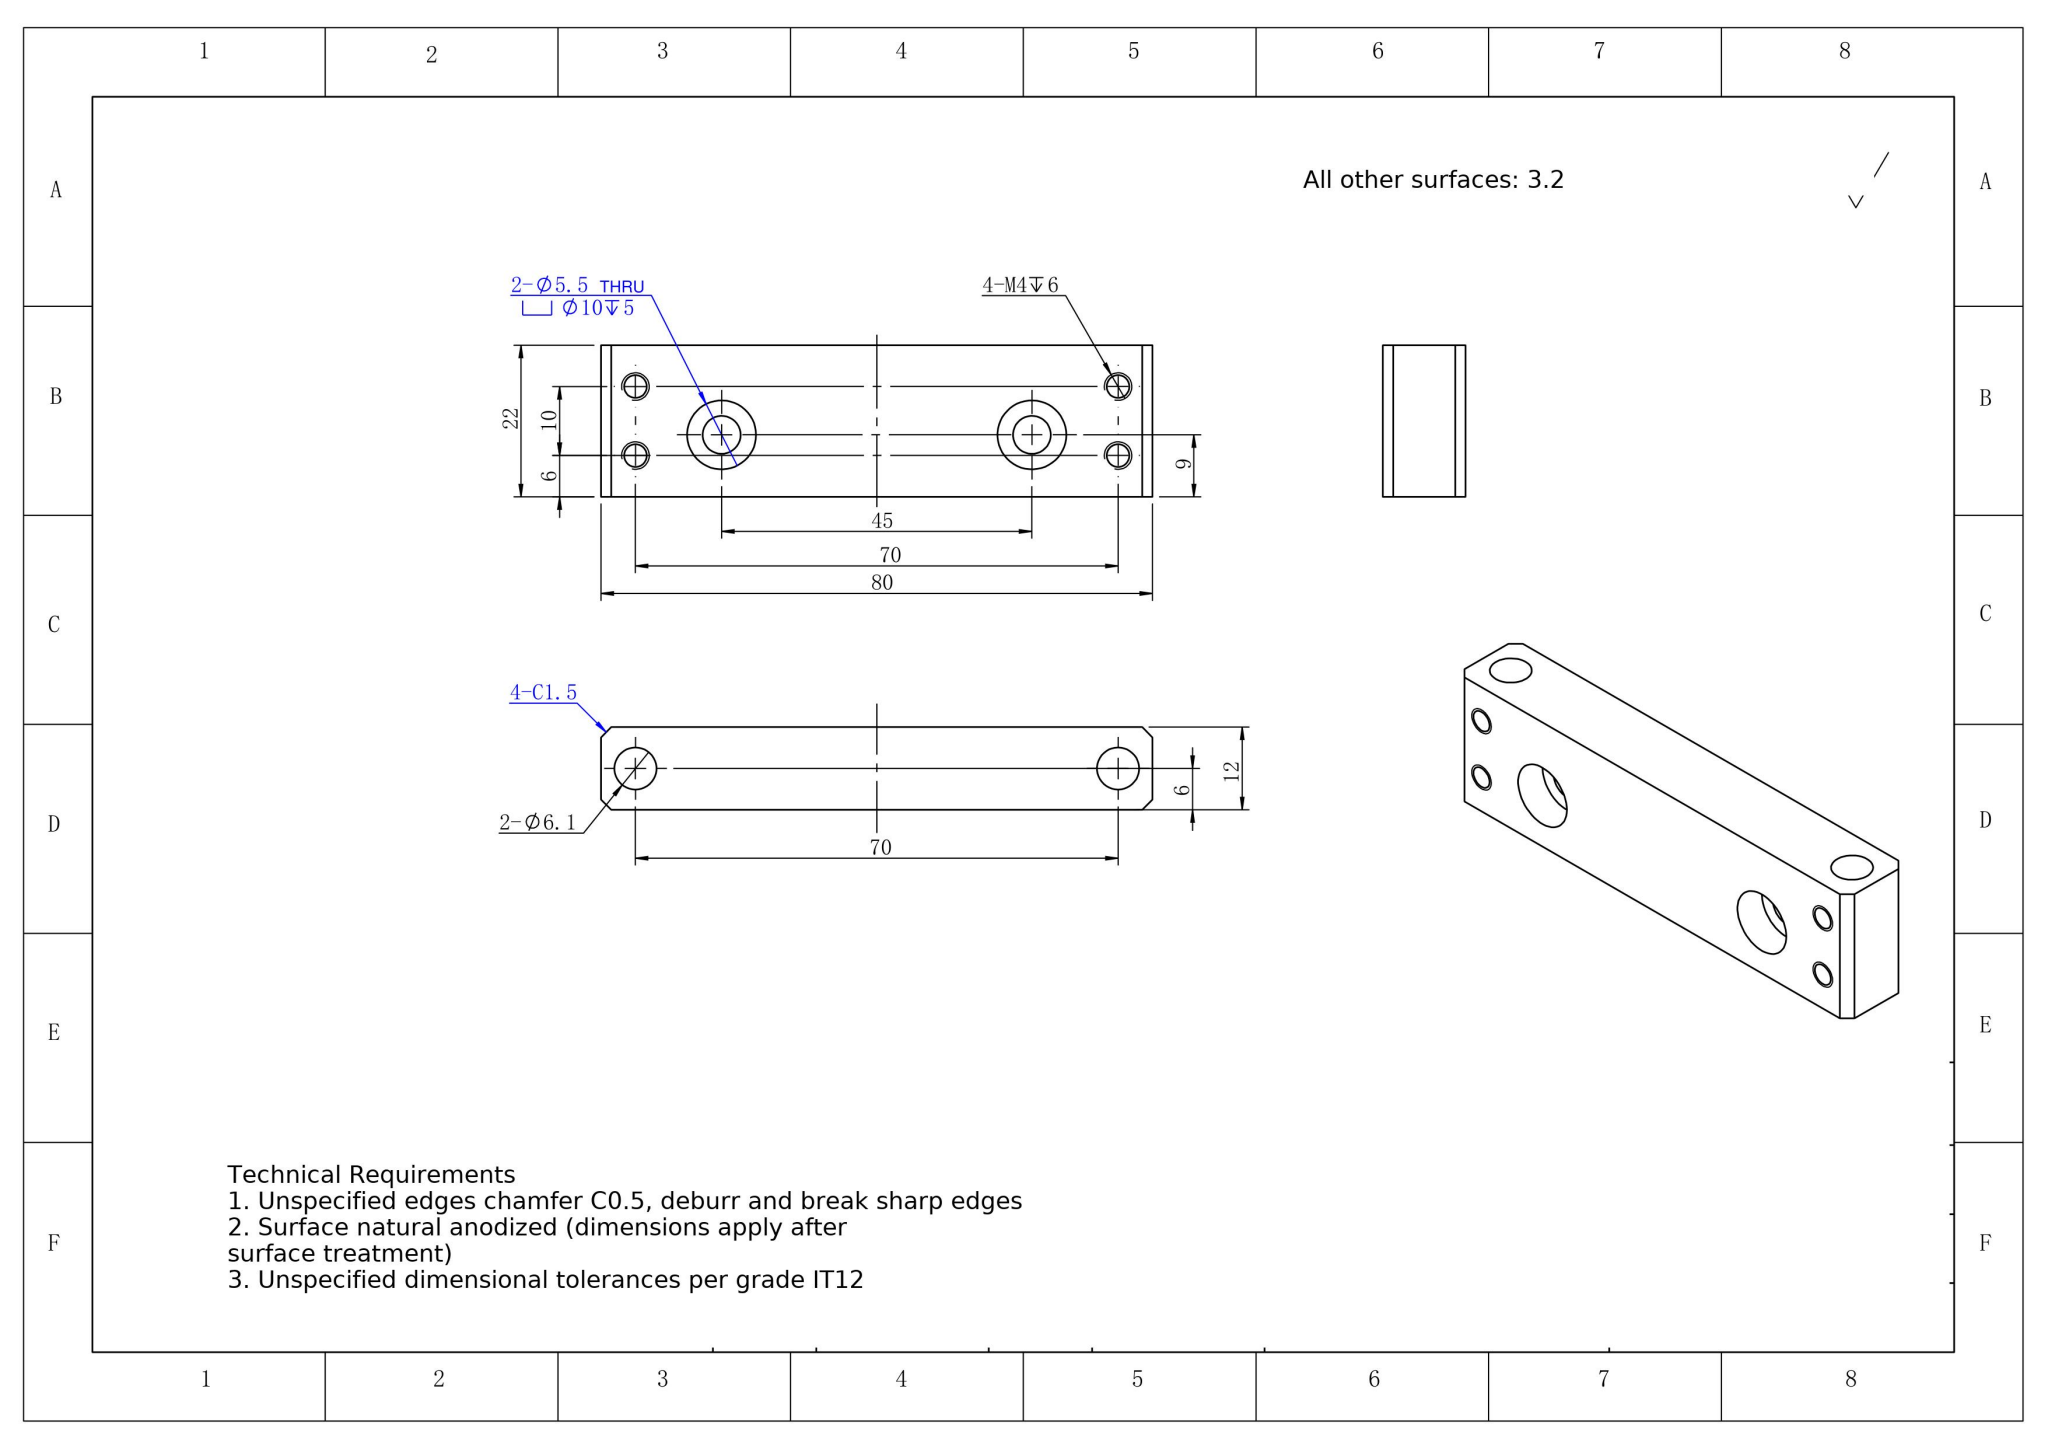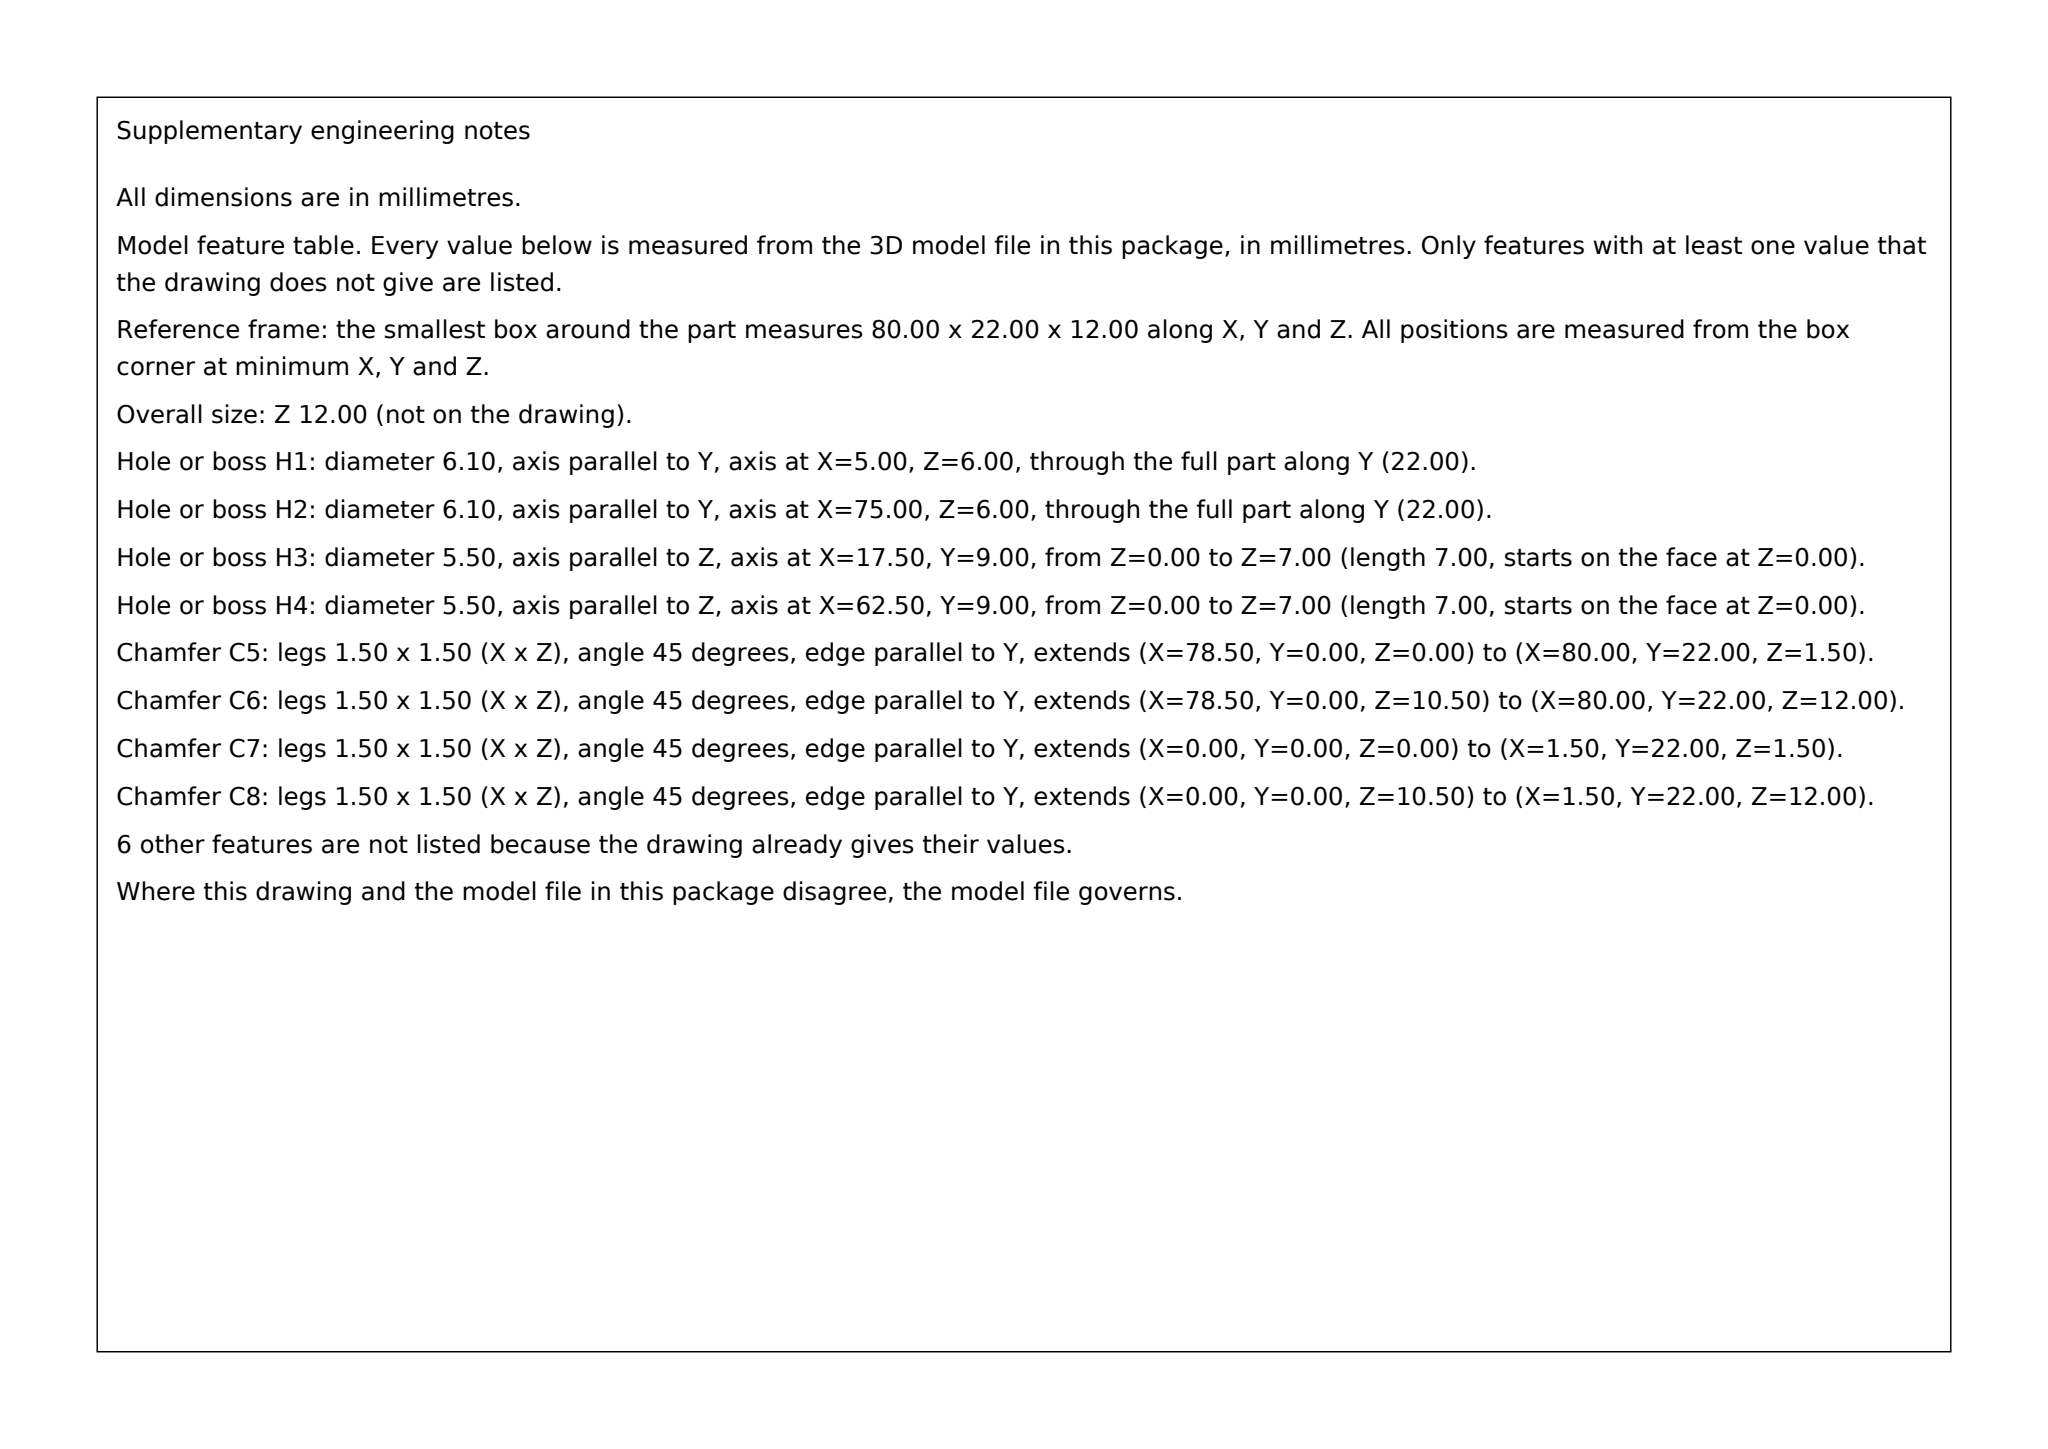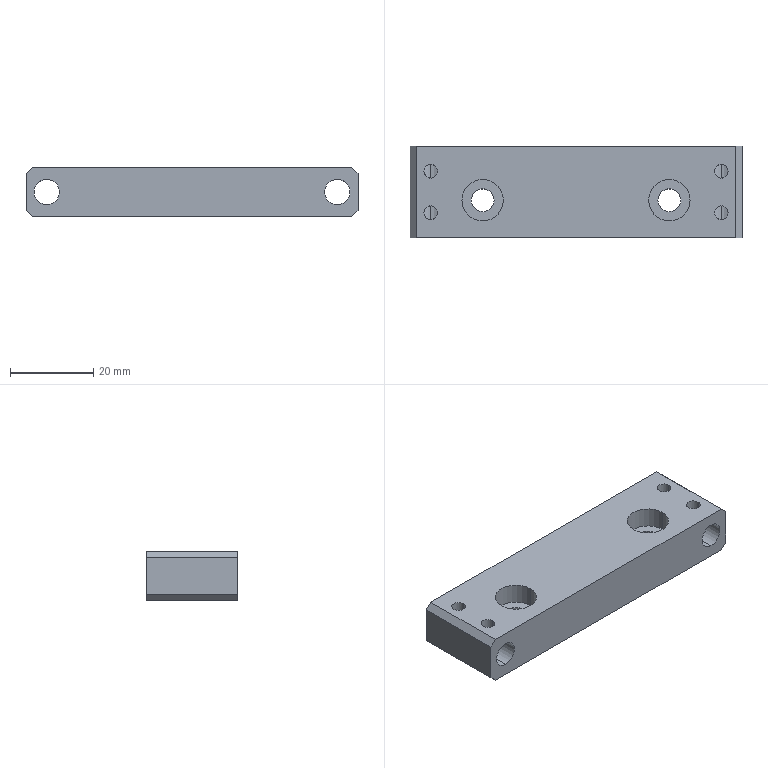Part | SolidWorks | mm | 1 solid | 32 faces | box 80 x 22 x 12 mm | volume 18512 mm3 | cylinder 20 | plane 12 | commonest cylinder face diameters 3.3 x8 10 x4 5.5 x4 6.1 x4
build123d program:
from build123d import *

# Parameters (mm, degrees)
SKETCH1_W                                         = 80
SKETCH1_H                                         = 22
BOSS_EXTRUDE1_DEPTH                               = 6
SKETCH3_R                                         = 3.05
CUT_EXTRUDE1_DEPTH                                = 47.043
M4_TAPPED_HOLE1_REACH                             = 49.202
M4_TAPPED_HOLE1_BORE_R                            = 1.65
HOLE_SIZE_ACCORDING_TO_HEXAGON_SOCKET_D           = 5.5
HOLE_SIZE_ACCORDING_TO_HEXAGON_SOCKET_CBORE_D     = 10
HOLE_SIZE_ACCORDING_TO_HEXAGON_SOCKET_CBORE_DEPTH = 5
CHAMFER1_SIZE                                     = 1.5


with BuildPart() as part:
    # Sketch1 → Boss-Extrude1 (new, symmetric)
    with BuildSketch(Plane.XY):
        with Locations((0, 11)):
            Rectangle(SKETCH1_W, SKETCH1_H)
    extrude(amount=BOSS_EXTRUDE1_DEPTH, both=True)

    # Sketch3 → Cut-Extrude1 (cut, through all)
    with BuildSketch(Plane(origin=(0, 22, 0), x_dir=(1, 0, 0), z_dir=(0, 1, 0))):
        with Locations(Location((-35, 0, 0), (0, 0, 270))):
            Circle(SKETCH3_R)
        with Locations(Location((35, 0, 0), (0, 0, 90))):
            Circle(SKETCH3_R)
    extrude(amount=-CUT_EXTRUDE1_DEPTH, mode=Mode.SUBTRACT)

    # M4 Tapped Hole1 bore → M4 Tapped Hole1 (cut, up to next)
    with BuildSketch(Plane.XY.offset(6), mode=Mode.PRIVATE) as m4_tapped_hole1_sk1:
        with Locations((-35, 16)):
            Circle(M4_TAPPED_HOLE1_BORE_R)
    m4_tapped_hole1_tool1 = extrude(m4_tapped_hole1_sk1.sketch, amount=-M4_TAPPED_HOLE1_REACH, mode=Mode.PRIVATE) & part.part
    # M4 Tapped Hole1 bore → M4 Tapped Hole1 (cut, up to next)
    with BuildSketch(Plane.XY.offset(6), mode=Mode.PRIVATE) as m4_tapped_hole1_sk2:
        with Locations((-35, 6)):
            Circle(M4_TAPPED_HOLE1_BORE_R)
    m4_tapped_hole1_tool2 = extrude(m4_tapped_hole1_sk2.sketch, amount=-M4_TAPPED_HOLE1_REACH, mode=Mode.PRIVATE) & part.part
    # M4 Tapped Hole1 bore → M4 Tapped Hole1 (cut, up to next)
    with BuildSketch(Plane.XY.offset(6), mode=Mode.PRIVATE) as m4_tapped_hole1_sk3:
        with Locations((35, 16)):
            Circle(M4_TAPPED_HOLE1_BORE_R)
    m4_tapped_hole1_tool3 = extrude(m4_tapped_hole1_sk3.sketch, amount=-M4_TAPPED_HOLE1_REACH, mode=Mode.PRIVATE) & part.part
    # M4 Tapped Hole1 bore → M4 Tapped Hole1 (cut, up to next)
    with BuildSketch(Plane.XY.offset(6), mode=Mode.PRIVATE) as m4_tapped_hole1_sk4:
        with Locations((35, 6)):
            Circle(M4_TAPPED_HOLE1_BORE_R)
    m4_tapped_hole1_tool4 = extrude(m4_tapped_hole1_sk4.sketch, amount=-M4_TAPPED_HOLE1_REACH, mode=Mode.PRIVATE) & part.part
    add(m4_tapped_hole1_tool1.solids().sort_by_distance((-35, 16, 6))[0], mode=Mode.SUBTRACT)
    add(m4_tapped_hole1_tool2.solids().sort_by_distance((-35, 6, 6))[0], mode=Mode.SUBTRACT)
    add(m4_tapped_hole1_tool3.solids().sort_by_distance((35, 16, 6))[0], mode=Mode.SUBTRACT)
    add(m4_tapped_hole1_tool4.solids().sort_by_distance((35, 6, 6))[0], mode=Mode.SUBTRACT)

    # Hole Size _ according to_ Hexagon Socket (through all)
    with Locations(Plane.XY.offset(6)):
        with Locations((-22.5, 9), (22.5, 9)):
            CounterBoreHole(HOLE_SIZE_ACCORDING_TO_HEXAGON_SOCKET_D / 2, HOLE_SIZE_ACCORDING_TO_HEXAGON_SOCKET_CBORE_D / 2, HOLE_SIZE_ACCORDING_TO_HEXAGON_SOCKET_CBORE_DEPTH)

    # Chamfer1
    chamfer1_edges = [part.edges().sort_by_distance(p)[0] for p in [
        (40, 11, 6),
        (-40, 11, 6),
        (40, 11, -6),
        (-40, 11, -6),
    ]]
    chamfer(chamfer1_edges, length=CHAMFER1_SIZE)


solid = part.part